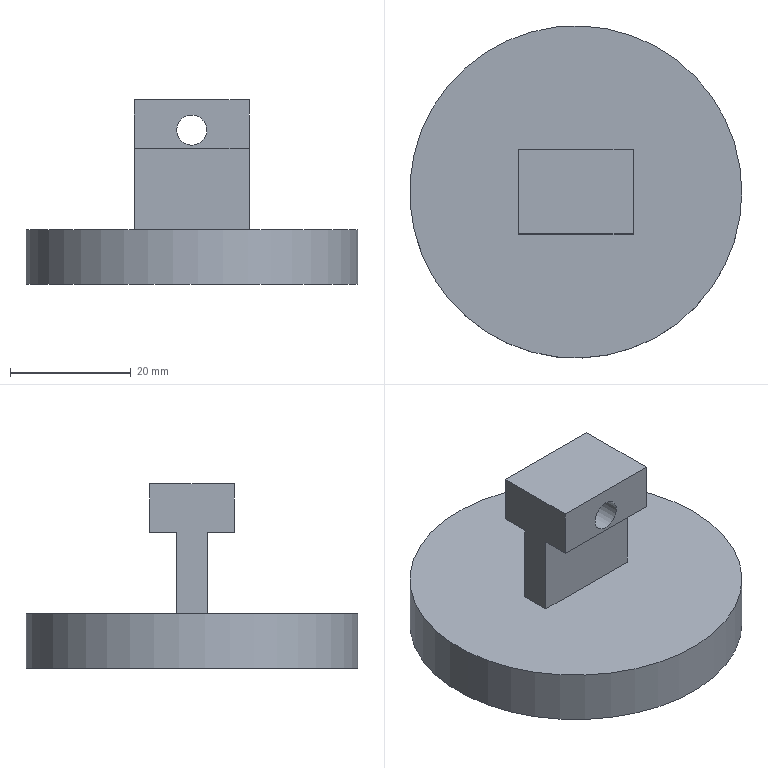Component | NX | STAMP_HOLDER | 1 solid | 13 faces | box 55 x 55 x 30.5 mm | volume 24518 mm3 | plane 11 | cylinder 2 | commonest cylinder face diameters 55 x1 5 x1
STEP:
#1=CARTESIAN_POINT('',(0.,0.,0.));
#2=DIRECTION('',(0.,0.,1.));
#3=DIRECTION('',(1.,0.,0.));
#4=AXIS2_PLACEMENT_3D('',#1,#2,#3);
#5=CARTESIAN_POINT('',(-107.476,-83.005,43.415));
#6=VERTEX_POINT('',#5);
#7=CARTESIAN_POINT('',(-134.976,-83.005,43.415));
#8=DIRECTION('',(0.,0.,-1.));
#9=DIRECTION('',(1.,0.,0.));
#10=AXIS2_PLACEMENT_3D('',#7,#8,#9);
#11=CIRCLE('',#10,27.5);
#12=CARTESIAN_POINT('',(-134.976,-83.005,43.415));
#13=DIRECTION('',(0.,0.,1.));
#14=DIRECTION('',(1.,0.,0.));
#15=AXIS2_PLACEMENT_3D('',#12,#13,#14);
#16=PLANE('',#15);
#17=CARTESIAN_POINT('',(27.5,0.));
#18=CARTESIAN_POINT('',(27.5,-47.631));
#19=CARTESIAN_POINT('',(-13.75,-23.816));
#20=CARTESIAN_POINT('',(-55.,-0.));
#21=CARTESIAN_POINT('',(-13.75,23.816));
#22=CARTESIAN_POINT('',(27.5,47.631));
#23=CARTESIAN_POINT('',(27.5,0.));
#24=(BOUNDED_CURVE()B_SPLINE_CURVE(2,(#17,#18,#19,#20,#21,#22,#23),.UNSPECIFIED.,.T.,.F.)B_SPLINE_CURVE_WITH_KNOTS((1,2,2,2,2,1),(-2.094,0.,2.094,4.189,6.283,8.378),.UNSPECIFIED.)CURVE()GEOMETRIC_REPRESENTATION_ITEM()RATIONAL_B_SPLINE_CURVE((1.,0.5,1.,0.5,1.,0.5,1.))REPRESENTATION_ITEM(''));
#25=(GEOMETRIC_REPRESENTATION_CONTEXT(2)PARAMETRIC_REPRESENTATION_CONTEXT()REPRESENTATION_CONTEXT('',''));
#26=DEFINITIONAL_REPRESENTATION('',(#24),#25);
#27=PCURVE('',#16,#26);
#28=CARTESIAN_POINT('',(-134.976,-83.005,34.415));
#29=DIRECTION('',(0.,0.,1.));
#30=DIRECTION('',(1.,0.,0.));
#31=AXIS2_PLACEMENT_3D('',#28,#29,#30);
#32=CYLINDRICAL_SURFACE('',#31,27.5);
#33=CARTESIAN_POINT('',(6.283,9.));
#34=DIRECTION('',(-1.,0.));
#35=VECTOR('',#34,1.);
#36=LINE('',#33,#35);
#37=(GEOMETRIC_REPRESENTATION_CONTEXT(2)PARAMETRIC_REPRESENTATION_CONTEXT()REPRESENTATION_CONTEXT('',''));
#38=DEFINITIONAL_REPRESENTATION('',(#36),#37);
#39=PCURVE('',#32,#38);
#40=SURFACE_CURVE('',#11,(#27,#39),.PCURVE_S1.);
#41=EDGE_CURVE('',#6,#6,#40,.T.);
#42=ORIENTED_EDGE('',*,*,#41,.F.);
#43=EDGE_LOOP('',(#42));
#44=FACE_BOUND('',#43,.T.);
#45=CARTESIAN_POINT('',(-125.476,-85.505,43.415));
#46=VERTEX_POINT('',#45);
#47=CARTESIAN_POINT('',(-144.476,-85.505,43.415));
#48=VERTEX_POINT('',#47);
#49=CARTESIAN_POINT('',(-125.476,-85.505,43.415));
#50=DIRECTION('',(-1.,0.,0.));
#51=VECTOR('',#50,1.);
#52=LINE('',#49,#51);
#53=CARTESIAN_POINT('',(9.5,-2.5));
#54=DIRECTION('',(-1.,0.));
#55=VECTOR('',#54,1.);
#56=LINE('',#53,#55);
#57=(GEOMETRIC_REPRESENTATION_CONTEXT(2)PARAMETRIC_REPRESENTATION_CONTEXT()REPRESENTATION_CONTEXT('',''));
#58=DEFINITIONAL_REPRESENTATION('',(#56),#57);
#59=PCURVE('',#16,#58);
#60=CARTESIAN_POINT('',(-125.476,-85.505,56.915));
#61=DIRECTION('',(0.,1.,-0.));
#62=DIRECTION('',(0.,0.,1.));
#63=AXIS2_PLACEMENT_3D('',#60,#61,#62);
#64=PLANE('',#63);
#65=CARTESIAN_POINT('',(-13.5,0.));
#66=DIRECTION('',(0.,-1.));
#67=VECTOR('',#66,1.);
#68=LINE('',#65,#67);
#69=(GEOMETRIC_REPRESENTATION_CONTEXT(2)PARAMETRIC_REPRESENTATION_CONTEXT()REPRESENTATION_CONTEXT('',''));
#70=DEFINITIONAL_REPRESENTATION('',(#68),#69);
#71=PCURVE('',#64,#70);
#72=SURFACE_CURVE('',#52,(#59,#71),.PCURVE_S1.);
#73=EDGE_CURVE('',#46,#48,#72,.T.);
#74=ORIENTED_EDGE('',*,*,#73,.T.);
#75=CARTESIAN_POINT('',(-144.476,-80.505,43.415));
#76=VERTEX_POINT('',#75);
#77=CARTESIAN_POINT('',(-144.476,-85.505,43.415));
#78=DIRECTION('',(0.,1.,0.));
#79=VECTOR('',#78,1.);
#80=LINE('',#77,#79);
#81=CARTESIAN_POINT('',(-9.5,-2.5));
#82=DIRECTION('',(0.,1.));
#83=VECTOR('',#82,1.);
#84=LINE('',#81,#83);
#85=(GEOMETRIC_REPRESENTATION_CONTEXT(2)PARAMETRIC_REPRESENTATION_CONTEXT()REPRESENTATION_CONTEXT('',''));
#86=DEFINITIONAL_REPRESENTATION('',(#84),#85);
#87=PCURVE('',#16,#86);
#88=CARTESIAN_POINT('',(-144.476,-83.005,34.415));
#89=DIRECTION('',(1.,0.,0.));
#90=DIRECTION('',(0.,0.,-1.));
#91=AXIS2_PLACEMENT_3D('',#88,#89,#90);
#92=PLANE('',#91);
#93=CARTESIAN_POINT('',(-9.,-2.5));
#94=DIRECTION('',(0.,1.));
#95=VECTOR('',#94,1.);
#96=LINE('',#93,#95);
#97=(GEOMETRIC_REPRESENTATION_CONTEXT(2)PARAMETRIC_REPRESENTATION_CONTEXT()REPRESENTATION_CONTEXT('',''));
#98=DEFINITIONAL_REPRESENTATION('',(#96),#97);
#99=PCURVE('',#92,#98);
#100=SURFACE_CURVE('',#80,(#87,#99),.PCURVE_S1.);
#101=EDGE_CURVE('',#48,#76,#100,.T.);
#102=ORIENTED_EDGE('',*,*,#101,.T.);
#103=CARTESIAN_POINT('',(-125.476,-80.505,43.415));
#104=VERTEX_POINT('',#103);
#105=CARTESIAN_POINT('',(-125.476,-80.505,43.415));
#106=DIRECTION('',(-1.,0.,0.));
#107=VECTOR('',#106,1.);
#108=LINE('',#105,#107);
#109=CARTESIAN_POINT('',(9.5,2.5));
#110=DIRECTION('',(-1.,0.));
#111=VECTOR('',#110,1.);
#112=LINE('',#109,#111);
#113=(GEOMETRIC_REPRESENTATION_CONTEXT(2)PARAMETRIC_REPRESENTATION_CONTEXT()REPRESENTATION_CONTEXT('',''));
#114=DEFINITIONAL_REPRESENTATION('',(#112),#113);
#115=PCURVE('',#16,#114);
#116=CARTESIAN_POINT('',(-125.476,-80.505,43.415));
#117=DIRECTION('',(0.,-1.,-0.));
#118=DIRECTION('',(0.,0.,-1.));
#119=AXIS2_PLACEMENT_3D('',#116,#117,#118);
#120=PLANE('',#119);
#121=CARTESIAN_POINT('',(0.,0.));
#122=DIRECTION('',(0.,-1.));
#123=VECTOR('',#122,1.);
#124=LINE('',#121,#123);
#125=(GEOMETRIC_REPRESENTATION_CONTEXT(2)PARAMETRIC_REPRESENTATION_CONTEXT()REPRESENTATION_CONTEXT('',''));
#126=DEFINITIONAL_REPRESENTATION('',(#124),#125);
#127=PCURVE('',#120,#126);
#128=SURFACE_CURVE('',#108,(#115,#127),.PCURVE_S1.);
#129=EDGE_CURVE('',#104,#76,#128,.T.);
#130=ORIENTED_EDGE('',*,*,#129,.F.);
#131=CARTESIAN_POINT('',(-125.476,-85.505,43.415));
#132=DIRECTION('',(0.,1.,0.));
#133=VECTOR('',#132,1.);
#134=LINE('',#131,#133);
#135=CARTESIAN_POINT('',(9.5,-2.5));
#136=DIRECTION('',(0.,1.));
#137=VECTOR('',#136,1.);
#138=LINE('',#135,#137);
#139=(GEOMETRIC_REPRESENTATION_CONTEXT(2)PARAMETRIC_REPRESENTATION_CONTEXT()REPRESENTATION_CONTEXT('',''));
#140=DEFINITIONAL_REPRESENTATION('',(#138),#139);
#141=PCURVE('',#16,#140);
#142=CARTESIAN_POINT('',(-125.476,-83.005,34.415));
#143=DIRECTION('',(1.,0.,0.));
#144=DIRECTION('',(0.,0.,-1.));
#145=AXIS2_PLACEMENT_3D('',#142,#143,#144);
#146=PLANE('',#145);
#147=CARTESIAN_POINT('',(-9.,-2.5));
#148=DIRECTION('',(0.,1.));
#149=VECTOR('',#148,1.);
#150=LINE('',#147,#149);
#151=(GEOMETRIC_REPRESENTATION_CONTEXT(2)PARAMETRIC_REPRESENTATION_CONTEXT()REPRESENTATION_CONTEXT('',''));
#152=DEFINITIONAL_REPRESENTATION('',(#150),#151);
#153=PCURVE('',#146,#152);
#154=SURFACE_CURVE('',#134,(#141,#153),.PCURVE_S1.);
#155=EDGE_CURVE('',#46,#104,#154,.T.);
#156=ORIENTED_EDGE('',*,*,#155,.F.);
#157=EDGE_LOOP('',(#74,#102,#130,#156));
#158=FACE_BOUND('',#157,.T.);
#159=ADVANCED_FACE('',(#44,#158),#16,.T.);
#160=CARTESIAN_POINT('',(-107.476,-83.005,34.415));
#161=VERTEX_POINT('',#160);
#162=CARTESIAN_POINT('',(-134.976,-83.005,34.415));
#163=DIRECTION('',(0.,0.,1.));
#164=DIRECTION('',(1.,0.,0.));
#165=AXIS2_PLACEMENT_3D('',#162,#163,#164);
#166=CIRCLE('',#165,27.5);
#167=CARTESIAN_POINT('',(-134.976,-83.005,34.415));
#168=DIRECTION('',(0.,0.,-1.));
#169=DIRECTION('',(-1.,0.,0.));
#170=AXIS2_PLACEMENT_3D('',#167,#168,#169);
#171=PLANE('',#170);
#172=CARTESIAN_POINT('',(-27.5,0.));
#173=CARTESIAN_POINT('',(-27.5,47.631));
#174=CARTESIAN_POINT('',(13.75,23.816));
#175=CARTESIAN_POINT('',(55.,0.));
#176=CARTESIAN_POINT('',(13.75,-23.816));
#177=CARTESIAN_POINT('',(-27.5,-47.631));
#178=CARTESIAN_POINT('',(-27.5,0.));
#179=(BOUNDED_CURVE()B_SPLINE_CURVE(2,(#172,#173,#174,#175,#176,#177,#178),.UNSPECIFIED.,.T.,.F.)B_SPLINE_CURVE_WITH_KNOTS((1,2,2,2,2,1),(-2.094,0.,2.094,4.189,6.283,8.378),.UNSPECIFIED.)CURVE()GEOMETRIC_REPRESENTATION_ITEM()RATIONAL_B_SPLINE_CURVE((1.,0.5,1.,0.5,1.,0.5,1.))REPRESENTATION_ITEM(''));
#180=(GEOMETRIC_REPRESENTATION_CONTEXT(2)PARAMETRIC_REPRESENTATION_CONTEXT()REPRESENTATION_CONTEXT('',''));
#181=DEFINITIONAL_REPRESENTATION('',(#179),#180);
#182=PCURVE('',#171,#181);
#183=CARTESIAN_POINT('',(0.,0.));
#184=DIRECTION('',(1.,0.));
#185=VECTOR('',#184,1.);
#186=LINE('',#183,#185);
#187=(GEOMETRIC_REPRESENTATION_CONTEXT(2)PARAMETRIC_REPRESENTATION_CONTEXT()REPRESENTATION_CONTEXT('',''));
#188=DEFINITIONAL_REPRESENTATION('',(#186),#187);
#189=PCURVE('',#32,#188);
#190=SURFACE_CURVE('',#166,(#182,#189),.PCURVE_S1.);
#191=EDGE_CURVE('',#161,#161,#190,.T.);
#192=ORIENTED_EDGE('',*,*,#191,.F.);
#193=EDGE_LOOP('',(#192));
#194=FACE_BOUND('',#193,.T.);
#195=ADVANCED_FACE('',(#194),#171,.T.);
#196=ORIENTED_EDGE('',*,*,#41,.T.);
#197=CARTESIAN_POINT('',(-107.476,-83.005,34.415));
#198=CARTESIAN_POINT('',(-107.476,-83.005,43.415));
#199=B_SPLINE_CURVE_WITH_KNOTS('',1,(#197,#198),.UNSPECIFIED.,.F.,.F.,(2,2),(0.,9.),.PIECEWISE_BEZIER_KNOTS.);
#200=CARTESIAN_POINT('',(0.,0.));
#201=DIRECTION('',(0.,1.));
#202=VECTOR('',#201,1.);
#203=LINE('',#200,#202);
#204=(GEOMETRIC_REPRESENTATION_CONTEXT(2)PARAMETRIC_REPRESENTATION_CONTEXT()REPRESENTATION_CONTEXT('',''));
#205=DEFINITIONAL_REPRESENTATION('',(#203),#204);
#206=PCURVE('',#32,#205);
#207=CARTESIAN_POINT('',(6.283,0.));
#208=DIRECTION('',(0.,1.));
#209=VECTOR('',#208,1.);
#210=LINE('',#207,#209);
#211=(GEOMETRIC_REPRESENTATION_CONTEXT(2)PARAMETRIC_REPRESENTATION_CONTEXT()REPRESENTATION_CONTEXT('',''));
#212=DEFINITIONAL_REPRESENTATION('',(#210),#211);
#213=PCURVE('',#32,#212);
#214=SEAM_CURVE('',#199,(#206,#213),.PCURVE_S1.);
#215=EDGE_CURVE('',#161,#6,#214,.T.);
#216=ORIENTED_EDGE('',*,*,#215,.F.);
#217=ORIENTED_EDGE('',*,*,#191,.T.);
#218=ORIENTED_EDGE('',*,*,#215,.T.);
#219=EDGE_LOOP('',(#196,#216,#217,#218));
#220=FACE_BOUND('',#219,.T.);
#221=ADVANCED_FACE('',(#220),#32,.T.);
#222=CARTESIAN_POINT('',(-134.976,-90.005,62.415));
#223=VERTEX_POINT('',#222);
#224=CARTESIAN_POINT('',(-134.976,-90.005,59.915));
#225=DIRECTION('',(0.,-1.,0.));
#226=DIRECTION('',(0.,0.,1.));
#227=AXIS2_PLACEMENT_3D('',#224,#225,#226);
#228=CIRCLE('',#227,2.5);
#229=CARTESIAN_POINT('',(-125.476,-90.005,64.915));
#230=DIRECTION('',(0.,1.,-0.));
#231=DIRECTION('',(0.,0.,1.));
#232=AXIS2_PLACEMENT_3D('',#229,#230,#231);
#233=PLANE('',#232);
#234=CARTESIAN_POINT('',(-2.5,-9.5));
#235=CARTESIAN_POINT('',(-2.5,-13.83));
#236=CARTESIAN_POINT('',(-6.25,-11.665));
#237=CARTESIAN_POINT('',(-10.,-9.5));
#238=CARTESIAN_POINT('',(-6.25,-7.335));
#239=CARTESIAN_POINT('',(-2.5,-5.17));
#240=CARTESIAN_POINT('',(-2.5,-9.5));
#241=(BOUNDED_CURVE()B_SPLINE_CURVE(2,(#234,#235,#236,#237,#238,#239,#240),.UNSPECIFIED.,.T.,.F.)B_SPLINE_CURVE_WITH_KNOTS((1,2,2,2,2,1),(-2.094,0.,2.094,4.189,6.283,8.378),.UNSPECIFIED.)CURVE()GEOMETRIC_REPRESENTATION_ITEM()RATIONAL_B_SPLINE_CURVE((1.,0.5,1.,0.5,1.,0.5,1.))REPRESENTATION_ITEM(''));
#242=(GEOMETRIC_REPRESENTATION_CONTEXT(2)PARAMETRIC_REPRESENTATION_CONTEXT()REPRESENTATION_CONTEXT('',''));
#243=DEFINITIONAL_REPRESENTATION('',(#241),#242);
#244=PCURVE('',#233,#243);
#245=CARTESIAN_POINT('',(-134.976,-92.505,59.915));
#246=DIRECTION('',(0.,1.,0.));
#247=DIRECTION('',(0.,0.,1.));
#248=AXIS2_PLACEMENT_3D('',#245,#246,#247);
#249=CYLINDRICAL_SURFACE('',#248,2.5);
#250=CARTESIAN_POINT('',(6.283,2.5));
#251=DIRECTION('',(-1.,0.));
#252=VECTOR('',#251,1.);
#253=LINE('',#250,#252);
#254=(GEOMETRIC_REPRESENTATION_CONTEXT(2)PARAMETRIC_REPRESENTATION_CONTEXT()REPRESENTATION_CONTEXT('',''));
#255=DEFINITIONAL_REPRESENTATION('',(#253),#254);
#256=PCURVE('',#249,#255);
#257=SURFACE_CURVE('',#228,(#244,#256),.PCURVE_S1.);
#258=EDGE_CURVE('',#223,#223,#257,.T.);
#259=ORIENTED_EDGE('',*,*,#258,.F.);
#260=EDGE_LOOP('',(#259));
#261=FACE_BOUND('',#260,.T.);
#262=CARTESIAN_POINT('',(-144.476,-90.005,64.915));
#263=VERTEX_POINT('',#262);
#264=CARTESIAN_POINT('',(-144.476,-90.005,56.915));
#265=VERTEX_POINT('',#264);
#266=CARTESIAN_POINT('',(-144.476,-90.005,64.915));
#267=DIRECTION('',(0.,-0.,-1.));
#268=VECTOR('',#267,1.);
#269=LINE('',#266,#268);
#270=CARTESIAN_POINT('',(0.,-19.));
#271=DIRECTION('',(-1.,0.));
#272=VECTOR('',#271,1.);
#273=LINE('',#270,#272);
#274=(GEOMETRIC_REPRESENTATION_CONTEXT(2)PARAMETRIC_REPRESENTATION_CONTEXT()REPRESENTATION_CONTEXT('',''));
#275=DEFINITIONAL_REPRESENTATION('',(#273),#274);
#276=PCURVE('',#233,#275);
#277=CARTESIAN_POINT('',(-30.5,-7.));
#278=DIRECTION('',(1.,-0.));
#279=VECTOR('',#278,1.);
#280=LINE('',#277,#279);
#281=(GEOMETRIC_REPRESENTATION_CONTEXT(2)PARAMETRIC_REPRESENTATION_CONTEXT()REPRESENTATION_CONTEXT('',''));
#282=DEFINITIONAL_REPRESENTATION('',(#280),#281);
#283=PCURVE('',#92,#282);
#284=SURFACE_CURVE('',#269,(#276,#283),.PCURVE_S1.);
#285=EDGE_CURVE('',#263,#265,#284,.T.);
#286=ORIENTED_EDGE('',*,*,#285,.T.);
#287=CARTESIAN_POINT('',(-125.476,-90.005,56.915));
#288=VERTEX_POINT('',#287);
#289=CARTESIAN_POINT('',(-125.476,-90.005,56.915));
#290=DIRECTION('',(-1.,0.,0.));
#291=VECTOR('',#290,1.);
#292=LINE('',#289,#291);
#293=CARTESIAN_POINT('',(-8.,0.));
#294=DIRECTION('',(0.,-1.));
#295=VECTOR('',#294,1.);
#296=LINE('',#293,#295);
#297=(GEOMETRIC_REPRESENTATION_CONTEXT(2)PARAMETRIC_REPRESENTATION_CONTEXT()REPRESENTATION_CONTEXT('',''));
#298=DEFINITIONAL_REPRESENTATION('',(#296),#297);
#299=PCURVE('',#233,#298);
#300=CARTESIAN_POINT('',(-125.476,-90.005,56.915));
#301=DIRECTION('',(0.,0.,1.));
#302=DIRECTION('',(1.,0.,0.));
#303=AXIS2_PLACEMENT_3D('',#300,#301,#302);
#304=PLANE('',#303);
#305=CARTESIAN_POINT('',(0.,0.));
#306=DIRECTION('',(-1.,0.));
#307=VECTOR('',#306,1.);
#308=LINE('',#305,#307);
#309=(GEOMETRIC_REPRESENTATION_CONTEXT(2)PARAMETRIC_REPRESENTATION_CONTEXT()REPRESENTATION_CONTEXT('',''));
#310=DEFINITIONAL_REPRESENTATION('',(#308),#309);
#311=PCURVE('',#304,#310);
#312=SURFACE_CURVE('',#292,(#299,#311),.PCURVE_S1.);
#313=EDGE_CURVE('',#288,#265,#312,.T.);
#314=ORIENTED_EDGE('',*,*,#313,.F.);
#315=CARTESIAN_POINT('',(-125.476,-90.005,64.915));
#316=VERTEX_POINT('',#315);
#317=CARTESIAN_POINT('',(-125.476,-90.005,64.915));
#318=DIRECTION('',(0.,-0.,-1.));
#319=VECTOR('',#318,1.);
#320=LINE('',#317,#319);
#321=CARTESIAN_POINT('',(0.,0.));
#322=DIRECTION('',(-1.,0.));
#323=VECTOR('',#322,1.);
#324=LINE('',#321,#323);
#325=(GEOMETRIC_REPRESENTATION_CONTEXT(2)PARAMETRIC_REPRESENTATION_CONTEXT()REPRESENTATION_CONTEXT('',''));
#326=DEFINITIONAL_REPRESENTATION('',(#324),#325);
#327=PCURVE('',#233,#326);
#328=CARTESIAN_POINT('',(-30.5,-7.));
#329=DIRECTION('',(1.,-0.));
#330=VECTOR('',#329,1.);
#331=LINE('',#328,#330);
#332=(GEOMETRIC_REPRESENTATION_CONTEXT(2)PARAMETRIC_REPRESENTATION_CONTEXT()REPRESENTATION_CONTEXT('',''));
#333=DEFINITIONAL_REPRESENTATION('',(#331),#332);
#334=PCURVE('',#146,#333);
#335=SURFACE_CURVE('',#320,(#327,#334),.PCURVE_S1.);
#336=EDGE_CURVE('',#316,#288,#335,.T.);
#337=ORIENTED_EDGE('',*,*,#336,.F.);
#338=CARTESIAN_POINT('',(-125.476,-90.005,64.915));
#339=DIRECTION('',(-1.,0.,0.));
#340=VECTOR('',#339,1.);
#341=LINE('',#338,#340);
#342=CARTESIAN_POINT('',(0.,0.));
#343=DIRECTION('',(0.,-1.));
#344=VECTOR('',#343,1.);
#345=LINE('',#342,#344);
#346=(GEOMETRIC_REPRESENTATION_CONTEXT(2)PARAMETRIC_REPRESENTATION_CONTEXT()REPRESENTATION_CONTEXT('',''));
#347=DEFINITIONAL_REPRESENTATION('',(#345),#346);
#348=PCURVE('',#233,#347);
#349=CARTESIAN_POINT('',(-125.476,-76.005,64.915));
#350=DIRECTION('',(0.,0.,-1.));
#351=DIRECTION('',(-1.,0.,0.));
#352=AXIS2_PLACEMENT_3D('',#349,#350,#351);
#353=PLANE('',#352);
#354=CARTESIAN_POINT('',(0.,-14.));
#355=DIRECTION('',(1.,0.));
#356=VECTOR('',#355,1.);
#357=LINE('',#354,#356);
#358=(GEOMETRIC_REPRESENTATION_CONTEXT(2)PARAMETRIC_REPRESENTATION_CONTEXT()REPRESENTATION_CONTEXT('',''));
#359=DEFINITIONAL_REPRESENTATION('',(#357),#358);
#360=PCURVE('',#353,#359);
#361=SURFACE_CURVE('',#341,(#348,#360),.PCURVE_S1.);
#362=EDGE_CURVE('',#316,#263,#361,.T.);
#363=ORIENTED_EDGE('',*,*,#362,.T.);
#364=EDGE_LOOP('',(#286,#314,#337,#363));
#365=FACE_BOUND('',#364,.T.);
#366=ADVANCED_FACE('',(#261,#365),#233,.F.);
#367=CARTESIAN_POINT('',(-144.476,-85.505,56.915));
#368=VERTEX_POINT('',#367);
#369=CARTESIAN_POINT('',(-144.476,-90.005,56.915));
#370=DIRECTION('',(0.,1.,0.));
#371=VECTOR('',#370,1.);
#372=LINE('',#369,#371);
#373=CARTESIAN_POINT('',(-19.,0.));
#374=DIRECTION('',(0.,1.));
#375=VECTOR('',#374,1.);
#376=LINE('',#373,#375);
#377=(GEOMETRIC_REPRESENTATION_CONTEXT(2)PARAMETRIC_REPRESENTATION_CONTEXT()REPRESENTATION_CONTEXT('',''));
#378=DEFINITIONAL_REPRESENTATION('',(#376),#377);
#379=PCURVE('',#304,#378);
#380=CARTESIAN_POINT('',(-22.5,-7.));
#381=DIRECTION('',(0.,1.));
#382=VECTOR('',#381,1.);
#383=LINE('',#380,#382);
#384=(GEOMETRIC_REPRESENTATION_CONTEXT(2)PARAMETRIC_REPRESENTATION_CONTEXT()REPRESENTATION_CONTEXT('',''));
#385=DEFINITIONAL_REPRESENTATION('',(#383),#384);
#386=PCURVE('',#92,#385);
#387=SURFACE_CURVE('',#372,(#379,#386),.PCURVE_S1.);
#388=EDGE_CURVE('',#265,#368,#387,.T.);
#389=ORIENTED_EDGE('',*,*,#388,.T.);
#390=CARTESIAN_POINT('',(-125.476,-85.505,56.915));
#391=VERTEX_POINT('',#390);
#392=CARTESIAN_POINT('',(-125.476,-85.505,56.915));
#393=DIRECTION('',(-1.,0.,0.));
#394=VECTOR('',#393,1.);
#395=LINE('',#392,#394);
#396=CARTESIAN_POINT('',(0.,4.5));
#397=DIRECTION('',(-1.,0.));
#398=VECTOR('',#397,1.);
#399=LINE('',#396,#398);
#400=(GEOMETRIC_REPRESENTATION_CONTEXT(2)PARAMETRIC_REPRESENTATION_CONTEXT()REPRESENTATION_CONTEXT('',''));
#401=DEFINITIONAL_REPRESENTATION('',(#399),#400);
#402=PCURVE('',#304,#401);
#403=CARTESIAN_POINT('',(0.,0.));
#404=DIRECTION('',(0.,-1.));
#405=VECTOR('',#404,1.);
#406=LINE('',#403,#405);
#407=(GEOMETRIC_REPRESENTATION_CONTEXT(2)PARAMETRIC_REPRESENTATION_CONTEXT()REPRESENTATION_CONTEXT('',''));
#408=DEFINITIONAL_REPRESENTATION('',(#406),#407);
#409=PCURVE('',#64,#408);
#410=SURFACE_CURVE('',#395,(#402,#409),.PCURVE_S1.);
#411=EDGE_CURVE('',#391,#368,#410,.T.);
#412=ORIENTED_EDGE('',*,*,#411,.F.);
#413=CARTESIAN_POINT('',(-125.476,-90.005,56.915));
#414=DIRECTION('',(0.,1.,0.));
#415=VECTOR('',#414,1.);
#416=LINE('',#413,#415);
#417=CARTESIAN_POINT('',(0.,0.));
#418=DIRECTION('',(0.,1.));
#419=VECTOR('',#418,1.);
#420=LINE('',#417,#419);
#421=(GEOMETRIC_REPRESENTATION_CONTEXT(2)PARAMETRIC_REPRESENTATION_CONTEXT()REPRESENTATION_CONTEXT('',''));
#422=DEFINITIONAL_REPRESENTATION('',(#420),#421);
#423=PCURVE('',#304,#422);
#424=CARTESIAN_POINT('',(-22.5,-7.));
#425=DIRECTION('',(0.,1.));
#426=VECTOR('',#425,1.);
#427=LINE('',#424,#426);
#428=(GEOMETRIC_REPRESENTATION_CONTEXT(2)PARAMETRIC_REPRESENTATION_CONTEXT()REPRESENTATION_CONTEXT('',''));
#429=DEFINITIONAL_REPRESENTATION('',(#427),#428);
#430=PCURVE('',#146,#429);
#431=SURFACE_CURVE('',#416,(#423,#430),.PCURVE_S1.);
#432=EDGE_CURVE('',#288,#391,#431,.T.);
#433=ORIENTED_EDGE('',*,*,#432,.F.);
#434=ORIENTED_EDGE('',*,*,#313,.T.);
#435=EDGE_LOOP('',(#389,#412,#433,#434));
#436=FACE_BOUND('',#435,.T.);
#437=ADVANCED_FACE('',(#436),#304,.F.);
#438=CARTESIAN_POINT('',(-144.476,-85.505,56.915));
#439=DIRECTION('',(0.,-0.,-1.));
#440=VECTOR('',#439,1.);
#441=LINE('',#438,#440);
#442=CARTESIAN_POINT('',(0.,-19.));
#443=DIRECTION('',(-1.,0.));
#444=VECTOR('',#443,1.);
#445=LINE('',#442,#444);
#446=(GEOMETRIC_REPRESENTATION_CONTEXT(2)PARAMETRIC_REPRESENTATION_CONTEXT()REPRESENTATION_CONTEXT('',''));
#447=DEFINITIONAL_REPRESENTATION('',(#445),#446);
#448=PCURVE('',#64,#447);
#449=CARTESIAN_POINT('',(-22.5,-2.5));
#450=DIRECTION('',(1.,-0.));
#451=VECTOR('',#450,1.);
#452=LINE('',#449,#451);
#453=(GEOMETRIC_REPRESENTATION_CONTEXT(2)PARAMETRIC_REPRESENTATION_CONTEXT()REPRESENTATION_CONTEXT('',''));
#454=DEFINITIONAL_REPRESENTATION('',(#452),#453);
#455=PCURVE('',#92,#454);
#456=SURFACE_CURVE('',#441,(#448,#455),.PCURVE_S1.);
#457=EDGE_CURVE('',#368,#48,#456,.T.);
#458=ORIENTED_EDGE('',*,*,#457,.T.);
#459=ORIENTED_EDGE('',*,*,#73,.F.);
#460=CARTESIAN_POINT('',(-125.476,-85.505,56.915));
#461=DIRECTION('',(0.,-0.,-1.));
#462=VECTOR('',#461,1.);
#463=LINE('',#460,#462);
#464=CARTESIAN_POINT('',(0.,0.));
#465=DIRECTION('',(-1.,0.));
#466=VECTOR('',#465,1.);
#467=LINE('',#464,#466);
#468=(GEOMETRIC_REPRESENTATION_CONTEXT(2)PARAMETRIC_REPRESENTATION_CONTEXT()REPRESENTATION_CONTEXT('',''));
#469=DEFINITIONAL_REPRESENTATION('',(#467),#468);
#470=PCURVE('',#64,#469);
#471=CARTESIAN_POINT('',(-22.5,-2.5));
#472=DIRECTION('',(1.,-0.));
#473=VECTOR('',#472,1.);
#474=LINE('',#471,#473);
#475=(GEOMETRIC_REPRESENTATION_CONTEXT(2)PARAMETRIC_REPRESENTATION_CONTEXT()REPRESENTATION_CONTEXT('',''));
#476=DEFINITIONAL_REPRESENTATION('',(#474),#475);
#477=PCURVE('',#146,#476);
#478=SURFACE_CURVE('',#463,(#470,#477),.PCURVE_S1.);
#479=EDGE_CURVE('',#391,#46,#478,.T.);
#480=ORIENTED_EDGE('',*,*,#479,.F.);
#481=ORIENTED_EDGE('',*,*,#411,.T.);
#482=EDGE_LOOP('',(#458,#459,#480,#481));
#483=FACE_BOUND('',#482,.T.);
#484=ADVANCED_FACE('',(#483),#64,.F.);
#485=CARTESIAN_POINT('',(-144.476,-80.505,56.915));
#486=VERTEX_POINT('',#485);
#487=CARTESIAN_POINT('',(-144.476,-80.505,43.415));
#488=DIRECTION('',(0.,-0.,1.));
#489=VECTOR('',#488,1.);
#490=LINE('',#487,#489);
#491=CARTESIAN_POINT('',(0.,-19.));
#492=DIRECTION('',(-1.,0.));
#493=VECTOR('',#492,1.);
#494=LINE('',#491,#493);
#495=(GEOMETRIC_REPRESENTATION_CONTEXT(2)PARAMETRIC_REPRESENTATION_CONTEXT()REPRESENTATION_CONTEXT('',''));
#496=DEFINITIONAL_REPRESENTATION('',(#494),#495);
#497=PCURVE('',#120,#496);
#498=CARTESIAN_POINT('',(-9.,2.5));
#499=DIRECTION('',(-1.,-0.));
#500=VECTOR('',#499,1.);
#501=LINE('',#498,#500);
#502=(GEOMETRIC_REPRESENTATION_CONTEXT(2)PARAMETRIC_REPRESENTATION_CONTEXT()REPRESENTATION_CONTEXT('',''));
#503=DEFINITIONAL_REPRESENTATION('',(#501),#502);
#504=PCURVE('',#92,#503);
#505=SURFACE_CURVE('',#490,(#497,#504),.PCURVE_S1.);
#506=EDGE_CURVE('',#76,#486,#505,.T.);
#507=ORIENTED_EDGE('',*,*,#506,.T.);
#508=CARTESIAN_POINT('',(-125.476,-80.505,56.915));
#509=VERTEX_POINT('',#508);
#510=CARTESIAN_POINT('',(-125.476,-80.505,56.915));
#511=DIRECTION('',(-1.,0.,0.));
#512=VECTOR('',#511,1.);
#513=LINE('',#510,#512);
#514=CARTESIAN_POINT('',(-13.5,0.));
#515=DIRECTION('',(0.,-1.));
#516=VECTOR('',#515,1.);
#517=LINE('',#514,#516);
#518=(GEOMETRIC_REPRESENTATION_CONTEXT(2)PARAMETRIC_REPRESENTATION_CONTEXT()REPRESENTATION_CONTEXT('',''));
#519=DEFINITIONAL_REPRESENTATION('',(#517),#518);
#520=PCURVE('',#120,#519);
#521=CARTESIAN_POINT('',(-125.476,-80.505,56.915));
#522=DIRECTION('',(0.,0.,1.));
#523=DIRECTION('',(1.,0.,0.));
#524=AXIS2_PLACEMENT_3D('',#521,#522,#523);
#525=PLANE('',#524);
#526=CARTESIAN_POINT('',(0.,0.));
#527=DIRECTION('',(-1.,0.));
#528=VECTOR('',#527,1.);
#529=LINE('',#526,#528);
#530=(GEOMETRIC_REPRESENTATION_CONTEXT(2)PARAMETRIC_REPRESENTATION_CONTEXT()REPRESENTATION_CONTEXT('',''));
#531=DEFINITIONAL_REPRESENTATION('',(#529),#530);
#532=PCURVE('',#525,#531);
#533=SURFACE_CURVE('',#513,(#520,#532),.PCURVE_S1.);
#534=EDGE_CURVE('',#509,#486,#533,.T.);
#535=ORIENTED_EDGE('',*,*,#534,.F.);
#536=CARTESIAN_POINT('',(-125.476,-80.505,43.415));
#537=DIRECTION('',(0.,-0.,1.));
#538=VECTOR('',#537,1.);
#539=LINE('',#536,#538);
#540=CARTESIAN_POINT('',(0.,0.));
#541=DIRECTION('',(-1.,0.));
#542=VECTOR('',#541,1.);
#543=LINE('',#540,#542);
#544=(GEOMETRIC_REPRESENTATION_CONTEXT(2)PARAMETRIC_REPRESENTATION_CONTEXT()REPRESENTATION_CONTEXT('',''));
#545=DEFINITIONAL_REPRESENTATION('',(#543),#544);
#546=PCURVE('',#120,#545);
#547=CARTESIAN_POINT('',(-9.,2.5));
#548=DIRECTION('',(-1.,-0.));
#549=VECTOR('',#548,1.);
#550=LINE('',#547,#549);
#551=(GEOMETRIC_REPRESENTATION_CONTEXT(2)PARAMETRIC_REPRESENTATION_CONTEXT()REPRESENTATION_CONTEXT('',''));
#552=DEFINITIONAL_REPRESENTATION('',(#550),#551);
#553=PCURVE('',#146,#552);
#554=SURFACE_CURVE('',#539,(#546,#553),.PCURVE_S1.);
#555=EDGE_CURVE('',#104,#509,#554,.T.);
#556=ORIENTED_EDGE('',*,*,#555,.F.);
#557=ORIENTED_EDGE('',*,*,#129,.T.);
#558=EDGE_LOOP('',(#507,#535,#556,#557));
#559=FACE_BOUND('',#558,.T.);
#560=ADVANCED_FACE('',(#559),#120,.F.);
#561=CARTESIAN_POINT('',(-144.476,-76.005,56.915));
#562=VERTEX_POINT('',#561);
#563=CARTESIAN_POINT('',(-144.476,-80.505,56.915));
#564=DIRECTION('',(0.,1.,0.));
#565=VECTOR('',#564,1.);
#566=LINE('',#563,#565);
#567=CARTESIAN_POINT('',(-19.,0.));
#568=DIRECTION('',(0.,1.));
#569=VECTOR('',#568,1.);
#570=LINE('',#567,#569);
#571=(GEOMETRIC_REPRESENTATION_CONTEXT(2)PARAMETRIC_REPRESENTATION_CONTEXT()REPRESENTATION_CONTEXT('',''));
#572=DEFINITIONAL_REPRESENTATION('',(#570),#571);
#573=PCURVE('',#525,#572);
#574=CARTESIAN_POINT('',(-22.5,2.5));
#575=DIRECTION('',(0.,1.));
#576=VECTOR('',#575,1.);
#577=LINE('',#574,#576);
#578=(GEOMETRIC_REPRESENTATION_CONTEXT(2)PARAMETRIC_REPRESENTATION_CONTEXT()REPRESENTATION_CONTEXT('',''));
#579=DEFINITIONAL_REPRESENTATION('',(#577),#578);
#580=PCURVE('',#92,#579);
#581=SURFACE_CURVE('',#566,(#573,#580),.PCURVE_S1.);
#582=EDGE_CURVE('',#486,#562,#581,.T.);
#583=ORIENTED_EDGE('',*,*,#582,.T.);
#584=CARTESIAN_POINT('',(-125.476,-76.005,56.915));
#585=VERTEX_POINT('',#584);
#586=CARTESIAN_POINT('',(-125.476,-76.005,56.915));
#587=DIRECTION('',(-1.,0.,0.));
#588=VECTOR('',#587,1.);
#589=LINE('',#586,#588);
#590=CARTESIAN_POINT('',(0.,4.5));
#591=DIRECTION('',(-1.,0.));
#592=VECTOR('',#591,1.);
#593=LINE('',#590,#592);
#594=(GEOMETRIC_REPRESENTATION_CONTEXT(2)PARAMETRIC_REPRESENTATION_CONTEXT()REPRESENTATION_CONTEXT('',''));
#595=DEFINITIONAL_REPRESENTATION('',(#593),#594);
#596=PCURVE('',#525,#595);
#597=CARTESIAN_POINT('',(-125.476,-76.005,56.915));
#598=DIRECTION('',(0.,-1.,-0.));
#599=DIRECTION('',(0.,0.,-1.));
#600=AXIS2_PLACEMENT_3D('',#597,#598,#599);
#601=PLANE('',#600);
#602=CARTESIAN_POINT('',(0.,0.));
#603=DIRECTION('',(0.,-1.));
#604=VECTOR('',#603,1.);
#605=LINE('',#602,#604);
#606=(GEOMETRIC_REPRESENTATION_CONTEXT(2)PARAMETRIC_REPRESENTATION_CONTEXT()REPRESENTATION_CONTEXT('',''));
#607=DEFINITIONAL_REPRESENTATION('',(#605),#606);
#608=PCURVE('',#601,#607);
#609=SURFACE_CURVE('',#589,(#596,#608),.PCURVE_S1.);
#610=EDGE_CURVE('',#585,#562,#609,.T.);
#611=ORIENTED_EDGE('',*,*,#610,.F.);
#612=CARTESIAN_POINT('',(-125.476,-80.505,56.915));
#613=DIRECTION('',(0.,1.,0.));
#614=VECTOR('',#613,1.);
#615=LINE('',#612,#614);
#616=CARTESIAN_POINT('',(0.,0.));
#617=DIRECTION('',(0.,1.));
#618=VECTOR('',#617,1.);
#619=LINE('',#616,#618);
#620=(GEOMETRIC_REPRESENTATION_CONTEXT(2)PARAMETRIC_REPRESENTATION_CONTEXT()REPRESENTATION_CONTEXT('',''));
#621=DEFINITIONAL_REPRESENTATION('',(#619),#620);
#622=PCURVE('',#525,#621);
#623=CARTESIAN_POINT('',(-22.5,2.5));
#624=DIRECTION('',(0.,1.));
#625=VECTOR('',#624,1.);
#626=LINE('',#623,#625);
#627=(GEOMETRIC_REPRESENTATION_CONTEXT(2)PARAMETRIC_REPRESENTATION_CONTEXT()REPRESENTATION_CONTEXT('',''));
#628=DEFINITIONAL_REPRESENTATION('',(#626),#627);
#629=PCURVE('',#146,#628);
#630=SURFACE_CURVE('',#615,(#622,#629),.PCURVE_S1.);
#631=EDGE_CURVE('',#509,#585,#630,.T.);
#632=ORIENTED_EDGE('',*,*,#631,.F.);
#633=ORIENTED_EDGE('',*,*,#534,.T.);
#634=EDGE_LOOP('',(#583,#611,#632,#633));
#635=FACE_BOUND('',#634,.T.);
#636=ADVANCED_FACE('',(#635),#525,.F.);
#637=CARTESIAN_POINT('',(-134.976,-76.005,57.415));
#638=VERTEX_POINT('',#637);
#639=CARTESIAN_POINT('',(-134.976,-76.005,62.415));
#640=VERTEX_POINT('',#639);
#641=CARTESIAN_POINT('',(-134.976,-76.005,59.915));
#642=DIRECTION('',(0.,1.,0.));
#643=DIRECTION('',(0.,0.,-1.));
#644=AXIS2_PLACEMENT_3D('',#641,#642,#643);
#645=CIRCLE('',#644,2.5);
#646=CARTESIAN_POINT('',(-0.5,-9.5));
#647=CARTESIAN_POINT('',(-0.5,-13.83));
#648=CARTESIAN_POINT('',(-4.25,-11.665));
#649=CARTESIAN_POINT('',(-8.,-9.5));
#650=CARTESIAN_POINT('',(-4.25,-7.335));
#651=CARTESIAN_POINT('',(-0.5,-5.17));
#652=CARTESIAN_POINT('',(-0.5,-9.5));
#653=(BOUNDED_CURVE()B_SPLINE_CURVE(2,(#646,#647,#648,#649,#650,#651,#652),.UNSPECIFIED.,.T.,.F.)B_SPLINE_CURVE_WITH_KNOTS((1,2,2,2,2,1),(-2.094,0.,2.094,4.189,6.283,8.378),.UNSPECIFIED.)CURVE()GEOMETRIC_REPRESENTATION_ITEM()RATIONAL_B_SPLINE_CURVE((1.,0.5,1.,0.5,1.,0.5,1.))REPRESENTATION_ITEM(''));
#654=(GEOMETRIC_REPRESENTATION_CONTEXT(2)PARAMETRIC_REPRESENTATION_CONTEXT()REPRESENTATION_CONTEXT('',''));
#655=DEFINITIONAL_REPRESENTATION('',(#653),#654);
#656=PCURVE('',#601,#655);
#657=CARTESIAN_POINT('',(3.142,16.5));
#658=DIRECTION('',(1.,0.));
#659=VECTOR('',#658,1.);
#660=LINE('',#657,#659);
#661=(GEOMETRIC_REPRESENTATION_CONTEXT(2)PARAMETRIC_REPRESENTATION_CONTEXT()REPRESENTATION_CONTEXT('',''));
#662=DEFINITIONAL_REPRESENTATION('',(#660),#661);
#663=PCURVE('',#249,#662);
#664=SURFACE_CURVE('',#645,(#656,#663),.PCURVE_S1.);
#665=EDGE_CURVE('',#638,#640,#664,.T.);
#666=ORIENTED_EDGE('',*,*,#665,.F.);
#667=CARTESIAN_POINT('',(-134.976,-76.005,59.915));
#668=DIRECTION('',(0.,1.,0.));
#669=DIRECTION('',(0.,0.,-1.));
#670=AXIS2_PLACEMENT_3D('',#667,#668,#669);
#671=CIRCLE('',#670,2.5);
#672=CARTESIAN_POINT('',(-0.5,-9.5));
#673=CARTESIAN_POINT('',(-0.5,-13.83));
#674=CARTESIAN_POINT('',(-4.25,-11.665));
#675=CARTESIAN_POINT('',(-8.,-9.5));
#676=CARTESIAN_POINT('',(-4.25,-7.335));
#677=CARTESIAN_POINT('',(-0.5,-5.17));
#678=CARTESIAN_POINT('',(-0.5,-9.5));
#679=(BOUNDED_CURVE()B_SPLINE_CURVE(2,(#672,#673,#674,#675,#676,#677,#678),.UNSPECIFIED.,.T.,.F.)B_SPLINE_CURVE_WITH_KNOTS((1,2,2,2,2,1),(-2.094,0.,2.094,4.189,6.283,8.378),.UNSPECIFIED.)CURVE()GEOMETRIC_REPRESENTATION_ITEM()RATIONAL_B_SPLINE_CURVE((1.,0.5,1.,0.5,1.,0.5,1.))REPRESENTATION_ITEM(''));
#680=(GEOMETRIC_REPRESENTATION_CONTEXT(2)PARAMETRIC_REPRESENTATION_CONTEXT()REPRESENTATION_CONTEXT('',''));
#681=DEFINITIONAL_REPRESENTATION('',(#679),#680);
#682=PCURVE('',#601,#681);
#683=CARTESIAN_POINT('',(-3.142,16.5));
#684=DIRECTION('',(1.,0.));
#685=VECTOR('',#684,1.);
#686=LINE('',#683,#685);
#687=(GEOMETRIC_REPRESENTATION_CONTEXT(2)PARAMETRIC_REPRESENTATION_CONTEXT()REPRESENTATION_CONTEXT('',''));
#688=DEFINITIONAL_REPRESENTATION('',(#686),#687);
#689=PCURVE('',#249,#688);
#690=SURFACE_CURVE('',#671,(#682,#689),.PCURVE_S1.);
#691=EDGE_CURVE('',#640,#638,#690,.T.);
#692=ORIENTED_EDGE('',*,*,#691,.F.);
#693=EDGE_LOOP('',(#666,#692));
#694=FACE_BOUND('',#693,.T.);
#695=CARTESIAN_POINT('',(-144.476,-76.005,64.915));
#696=VERTEX_POINT('',#695);
#697=CARTESIAN_POINT('',(-144.476,-76.005,56.915));
#698=DIRECTION('',(0.,-0.,1.));
#699=VECTOR('',#698,1.);
#700=LINE('',#697,#699);
#701=CARTESIAN_POINT('',(0.,-19.));
#702=DIRECTION('',(-1.,0.));
#703=VECTOR('',#702,1.);
#704=LINE('',#701,#703);
#705=(GEOMETRIC_REPRESENTATION_CONTEXT(2)PARAMETRIC_REPRESENTATION_CONTEXT()REPRESENTATION_CONTEXT('',''));
#706=DEFINITIONAL_REPRESENTATION('',(#704),#705);
#707=PCURVE('',#601,#706);
#708=CARTESIAN_POINT('',(-22.5,7.));
#709=DIRECTION('',(-1.,-0.));
#710=VECTOR('',#709,1.);
#711=LINE('',#708,#710);
#712=(GEOMETRIC_REPRESENTATION_CONTEXT(2)PARAMETRIC_REPRESENTATION_CONTEXT()REPRESENTATION_CONTEXT('',''));
#713=DEFINITIONAL_REPRESENTATION('',(#711),#712);
#714=PCURVE('',#92,#713);
#715=SURFACE_CURVE('',#700,(#707,#714),.PCURVE_S1.);
#716=EDGE_CURVE('',#562,#696,#715,.T.);
#717=ORIENTED_EDGE('',*,*,#716,.T.);
#718=CARTESIAN_POINT('',(-125.476,-76.005,64.915));
#719=VERTEX_POINT('',#718);
#720=CARTESIAN_POINT('',(-125.476,-76.005,64.915));
#721=DIRECTION('',(-1.,0.,0.));
#722=VECTOR('',#721,1.);
#723=LINE('',#720,#722);
#724=CARTESIAN_POINT('',(-8.,0.));
#725=DIRECTION('',(0.,-1.));
#726=VECTOR('',#725,1.);
#727=LINE('',#724,#726);
#728=(GEOMETRIC_REPRESENTATION_CONTEXT(2)PARAMETRIC_REPRESENTATION_CONTEXT()REPRESENTATION_CONTEXT('',''));
#729=DEFINITIONAL_REPRESENTATION('',(#727),#728);
#730=PCURVE('',#601,#729);
#731=CARTESIAN_POINT('',(0.,0.));
#732=DIRECTION('',(1.,0.));
#733=VECTOR('',#732,1.);
#734=LINE('',#731,#733);
#735=(GEOMETRIC_REPRESENTATION_CONTEXT(2)PARAMETRIC_REPRESENTATION_CONTEXT()REPRESENTATION_CONTEXT('',''));
#736=DEFINITIONAL_REPRESENTATION('',(#734),#735);
#737=PCURVE('',#353,#736);
#738=SURFACE_CURVE('',#723,(#730,#737),.PCURVE_S1.);
#739=EDGE_CURVE('',#719,#696,#738,.T.);
#740=ORIENTED_EDGE('',*,*,#739,.F.);
#741=CARTESIAN_POINT('',(-125.476,-76.005,56.915));
#742=DIRECTION('',(0.,-0.,1.));
#743=VECTOR('',#742,1.);
#744=LINE('',#741,#743);
#745=CARTESIAN_POINT('',(0.,0.));
#746=DIRECTION('',(-1.,0.));
#747=VECTOR('',#746,1.);
#748=LINE('',#745,#747);
#749=(GEOMETRIC_REPRESENTATION_CONTEXT(2)PARAMETRIC_REPRESENTATION_CONTEXT()REPRESENTATION_CONTEXT('',''));
#750=DEFINITIONAL_REPRESENTATION('',(#748),#749);
#751=PCURVE('',#601,#750);
#752=CARTESIAN_POINT('',(-22.5,7.));
#753=DIRECTION('',(-1.,-0.));
#754=VECTOR('',#753,1.);
#755=LINE('',#752,#754);
#756=(GEOMETRIC_REPRESENTATION_CONTEXT(2)PARAMETRIC_REPRESENTATION_CONTEXT()REPRESENTATION_CONTEXT('',''));
#757=DEFINITIONAL_REPRESENTATION('',(#755),#756);
#758=PCURVE('',#146,#757);
#759=SURFACE_CURVE('',#744,(#751,#758),.PCURVE_S1.);
#760=EDGE_CURVE('',#585,#719,#759,.T.);
#761=ORIENTED_EDGE('',*,*,#760,.F.);
#762=ORIENTED_EDGE('',*,*,#610,.T.);
#763=EDGE_LOOP('',(#717,#740,#761,#762));
#764=FACE_BOUND('',#763,.T.);
#765=ADVANCED_FACE('',(#694,#764),#601,.F.);
#766=CARTESIAN_POINT('',(-144.476,-76.005,64.915));
#767=DIRECTION('',(0.,-1.,0.));
#768=VECTOR('',#767,1.);
#769=LINE('',#766,#768);
#770=CARTESIAN_POINT('',(19.,0.));
#771=DIRECTION('',(0.,-1.));
#772=VECTOR('',#771,1.);
#773=LINE('',#770,#772);
#774=(GEOMETRIC_REPRESENTATION_CONTEXT(2)PARAMETRIC_REPRESENTATION_CONTEXT()REPRESENTATION_CONTEXT('',''));
#775=DEFINITIONAL_REPRESENTATION('',(#773),#774);
#776=PCURVE('',#353,#775);
#777=CARTESIAN_POINT('',(-30.5,7.));
#778=DIRECTION('',(0.,-1.));
#779=VECTOR('',#778,1.);
#780=LINE('',#777,#779);
#781=(GEOMETRIC_REPRESENTATION_CONTEXT(2)PARAMETRIC_REPRESENTATION_CONTEXT()REPRESENTATION_CONTEXT('',''));
#782=DEFINITIONAL_REPRESENTATION('',(#780),#781);
#783=PCURVE('',#92,#782);
#784=SURFACE_CURVE('',#769,(#776,#783),.PCURVE_S1.);
#785=EDGE_CURVE('',#696,#263,#784,.T.);
#786=ORIENTED_EDGE('',*,*,#785,.T.);
#787=ORIENTED_EDGE('',*,*,#362,.F.);
#788=CARTESIAN_POINT('',(-125.476,-76.005,64.915));
#789=DIRECTION('',(0.,-1.,0.));
#790=VECTOR('',#789,1.);
#791=LINE('',#788,#790);
#792=CARTESIAN_POINT('',(0.,0.));
#793=DIRECTION('',(0.,-1.));
#794=VECTOR('',#793,1.);
#795=LINE('',#792,#794);
#796=(GEOMETRIC_REPRESENTATION_CONTEXT(2)PARAMETRIC_REPRESENTATION_CONTEXT()REPRESENTATION_CONTEXT('',''));
#797=DEFINITIONAL_REPRESENTATION('',(#795),#796);
#798=PCURVE('',#353,#797);
#799=CARTESIAN_POINT('',(-30.5,7.));
#800=DIRECTION('',(0.,-1.));
#801=VECTOR('',#800,1.);
#802=LINE('',#799,#801);
#803=(GEOMETRIC_REPRESENTATION_CONTEXT(2)PARAMETRIC_REPRESENTATION_CONTEXT()REPRESENTATION_CONTEXT('',''));
#804=DEFINITIONAL_REPRESENTATION('',(#802),#803);
#805=PCURVE('',#146,#804);
#806=SURFACE_CURVE('',#791,(#798,#805),.PCURVE_S1.);
#807=EDGE_CURVE('',#719,#316,#806,.T.);
#808=ORIENTED_EDGE('',*,*,#807,.F.);
#809=ORIENTED_EDGE('',*,*,#739,.T.);
#810=EDGE_LOOP('',(#786,#787,#808,#809));
#811=FACE_BOUND('',#810,.T.);
#812=ADVANCED_FACE('',(#811),#353,.F.);
#813=ORIENTED_EDGE('',*,*,#336,.T.);
#814=ORIENTED_EDGE('',*,*,#432,.T.);
#815=ORIENTED_EDGE('',*,*,#479,.T.);
#816=ORIENTED_EDGE('',*,*,#155,.T.);
#817=ORIENTED_EDGE('',*,*,#555,.T.);
#818=ORIENTED_EDGE('',*,*,#631,.T.);
#819=ORIENTED_EDGE('',*,*,#760,.T.);
#820=ORIENTED_EDGE('',*,*,#807,.T.);
#821=EDGE_LOOP('',(#813,#814,#815,#816,#817,#818,#819,#820));
#822=FACE_BOUND('',#821,.T.);
#823=ADVANCED_FACE('',(#822),#146,.T.);
#824=ORIENTED_EDGE('',*,*,#285,.F.);
#825=ORIENTED_EDGE('',*,*,#785,.F.);
#826=ORIENTED_EDGE('',*,*,#716,.F.);
#827=ORIENTED_EDGE('',*,*,#582,.F.);
#828=ORIENTED_EDGE('',*,*,#506,.F.);
#829=ORIENTED_EDGE('',*,*,#101,.F.);
#830=ORIENTED_EDGE('',*,*,#457,.F.);
#831=ORIENTED_EDGE('',*,*,#388,.F.);
#832=EDGE_LOOP('',(#824,#825,#826,#827,#828,#829,#830,#831));
#833=FACE_BOUND('',#832,.T.);
#834=ADVANCED_FACE('',(#833),#92,.F.);
#835=ORIENTED_EDGE('',*,*,#691,.F.);
#836=CARTESIAN_POINT('',(-134.976,-90.005,62.415));
#837=CARTESIAN_POINT('',(-134.976,-76.005,62.415));
#838=B_SPLINE_CURVE_WITH_KNOTS('',1,(#836,#837),.UNSPECIFIED.,.F.,.F.,(2,2),(2.5,16.5),.PIECEWISE_BEZIER_KNOTS.);
#839=CARTESIAN_POINT('',(0.,0.));
#840=DIRECTION('',(0.,1.));
#841=VECTOR('',#840,1.);
#842=LINE('',#839,#841);
#843=(GEOMETRIC_REPRESENTATION_CONTEXT(2)PARAMETRIC_REPRESENTATION_CONTEXT()REPRESENTATION_CONTEXT('',''));
#844=DEFINITIONAL_REPRESENTATION('',(#842),#843);
#845=PCURVE('',#249,#844);
#846=CARTESIAN_POINT('',(6.283,0.));
#847=DIRECTION('',(0.,1.));
#848=VECTOR('',#847,1.);
#849=LINE('',#846,#848);
#850=(GEOMETRIC_REPRESENTATION_CONTEXT(2)PARAMETRIC_REPRESENTATION_CONTEXT()REPRESENTATION_CONTEXT('',''));
#851=DEFINITIONAL_REPRESENTATION('',(#849),#850);
#852=PCURVE('',#249,#851);
#853=SEAM_CURVE('',#838,(#845,#852),.PCURVE_S1.);
#854=EDGE_CURVE('',#223,#640,#853,.T.);
#855=ORIENTED_EDGE('',*,*,#854,.F.);
#856=ORIENTED_EDGE('',*,*,#258,.F.);
#857=ORIENTED_EDGE('',*,*,#854,.T.);
#858=ORIENTED_EDGE('',*,*,#665,.F.);
#859=EDGE_LOOP('',(#835,#855,#856,#857,#858));
#860=FACE_BOUND('',#859,.F.);
#861=ADVANCED_FACE('',(#860),#249,.F.);
#862=CLOSED_SHELL('',(#159,#195,#221,#366,#437,#484,#560,#636,#765,#812,#823,#834,#861));
#863=MANIFOLD_SOLID_BREP('',#862);
#864=(LENGTH_UNIT()NAMED_UNIT(*)SI_UNIT(.MILLI.,.METRE.));
#865=UNCERTAINTY_MEASURE_WITH_UNIT(LENGTH_MEASURE(0.000002),#864,'','');
#866=(NAMED_UNIT(*)PLANE_ANGLE_UNIT()SI_UNIT($,.RADIAN.));
#867=(NAMED_UNIT(*)SI_UNIT($,.STERADIAN.)SOLID_ANGLE_UNIT());
#868=(GEOMETRIC_REPRESENTATION_CONTEXT(3)GLOBAL_UNCERTAINTY_ASSIGNED_CONTEXT((#865))GLOBAL_UNIT_ASSIGNED_CONTEXT((#864,#866,#867))REPRESENTATION_CONTEXT('',''));
#869=ADVANCED_BREP_SHAPE_REPRESENTATION('',(#4,#863),#868);